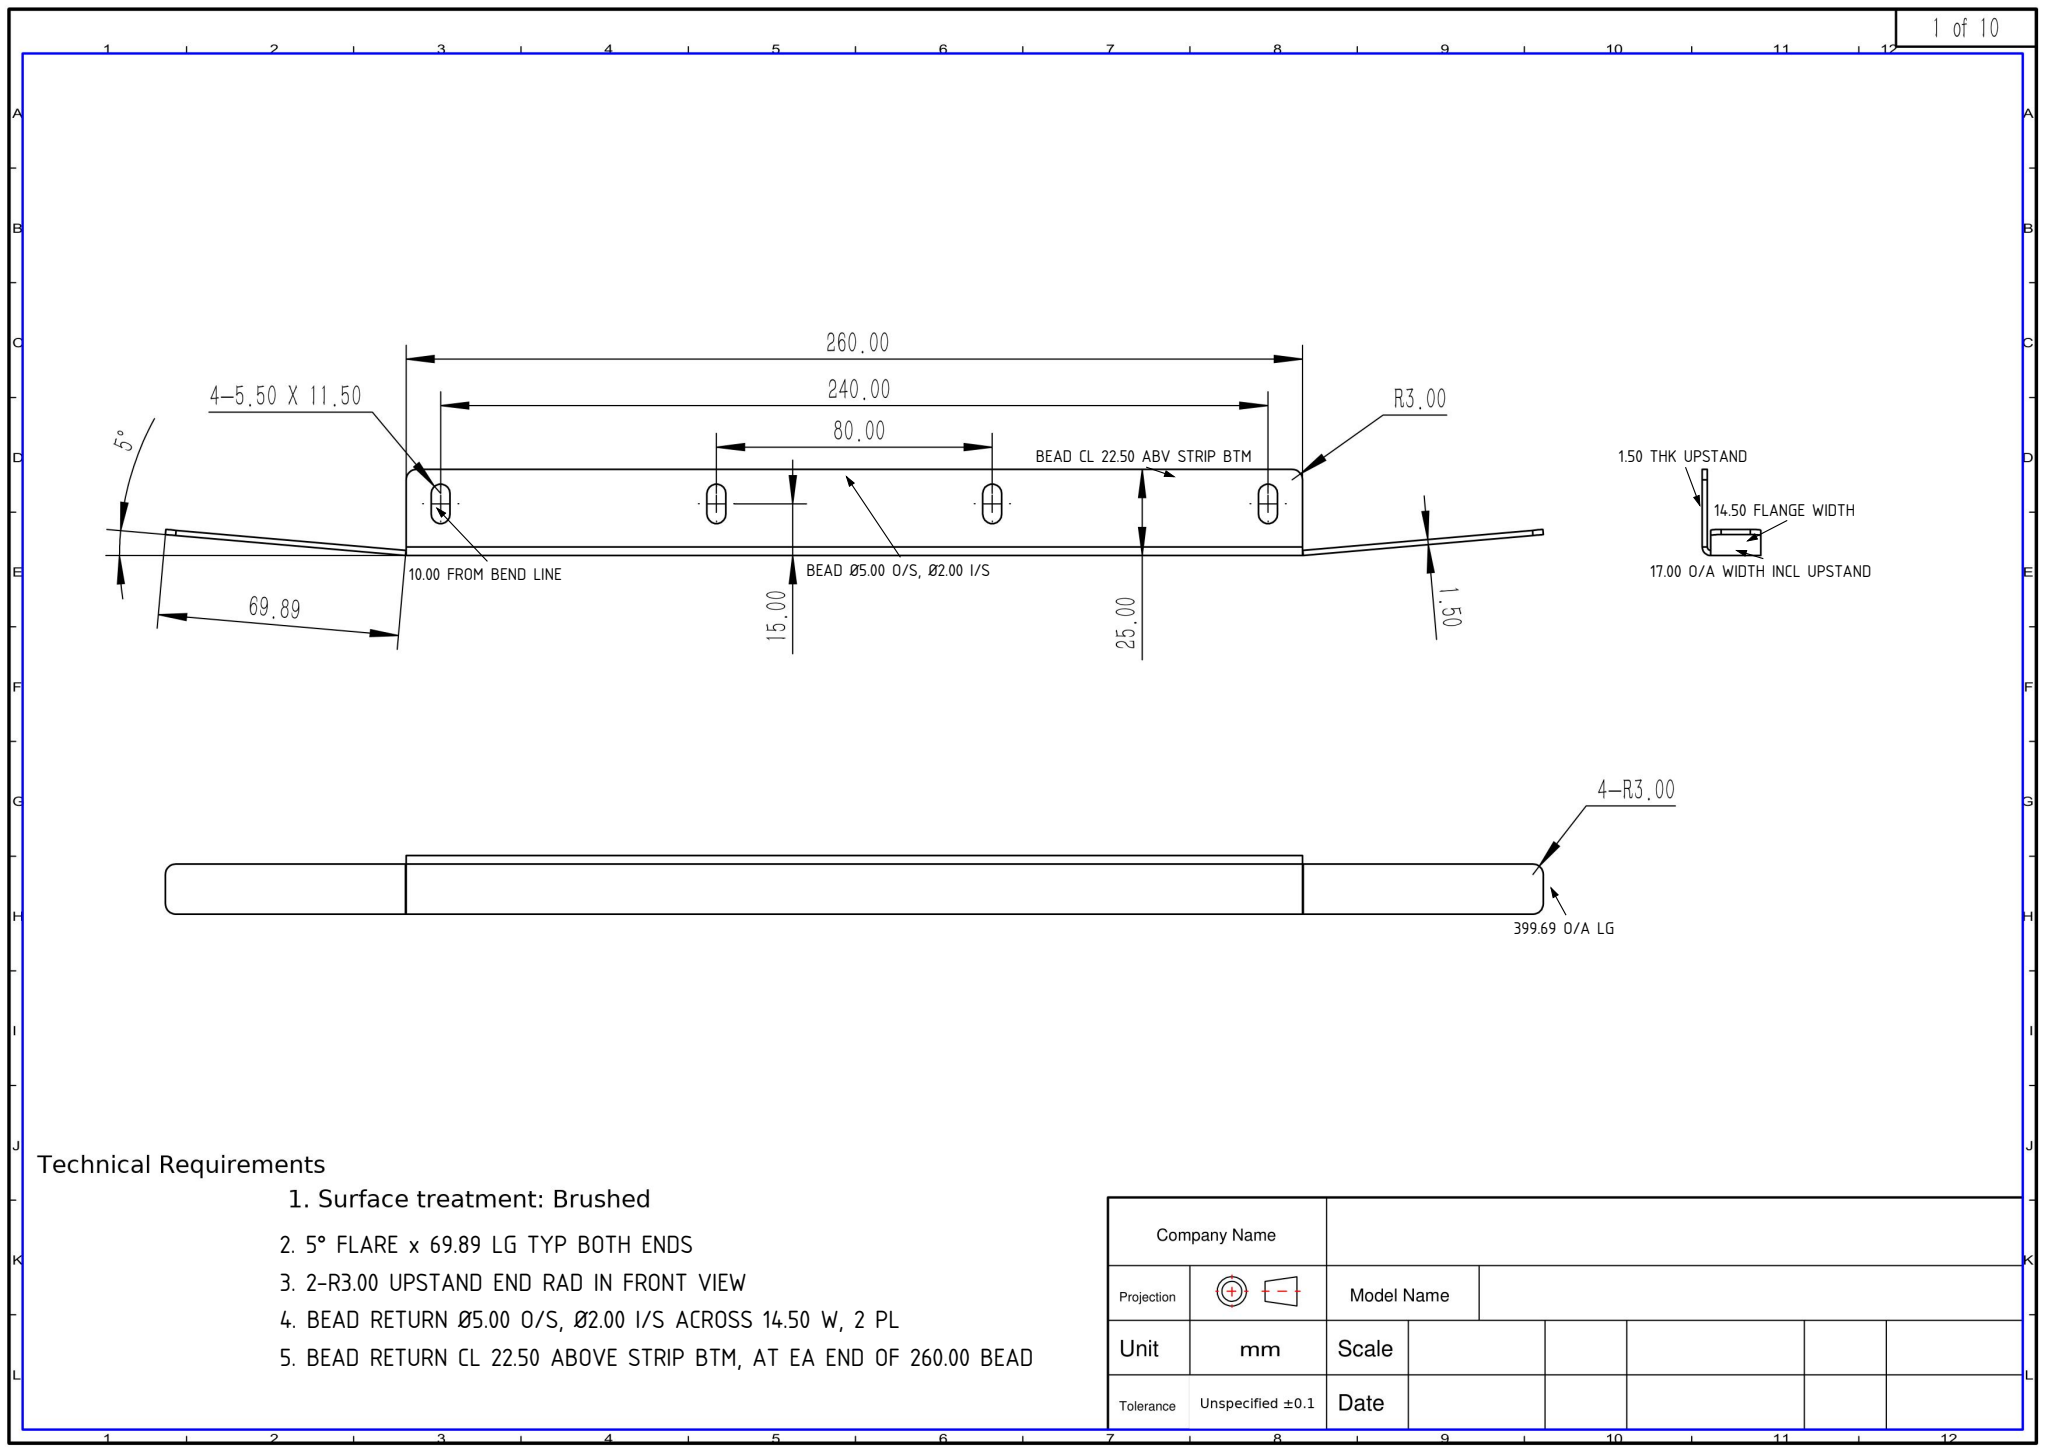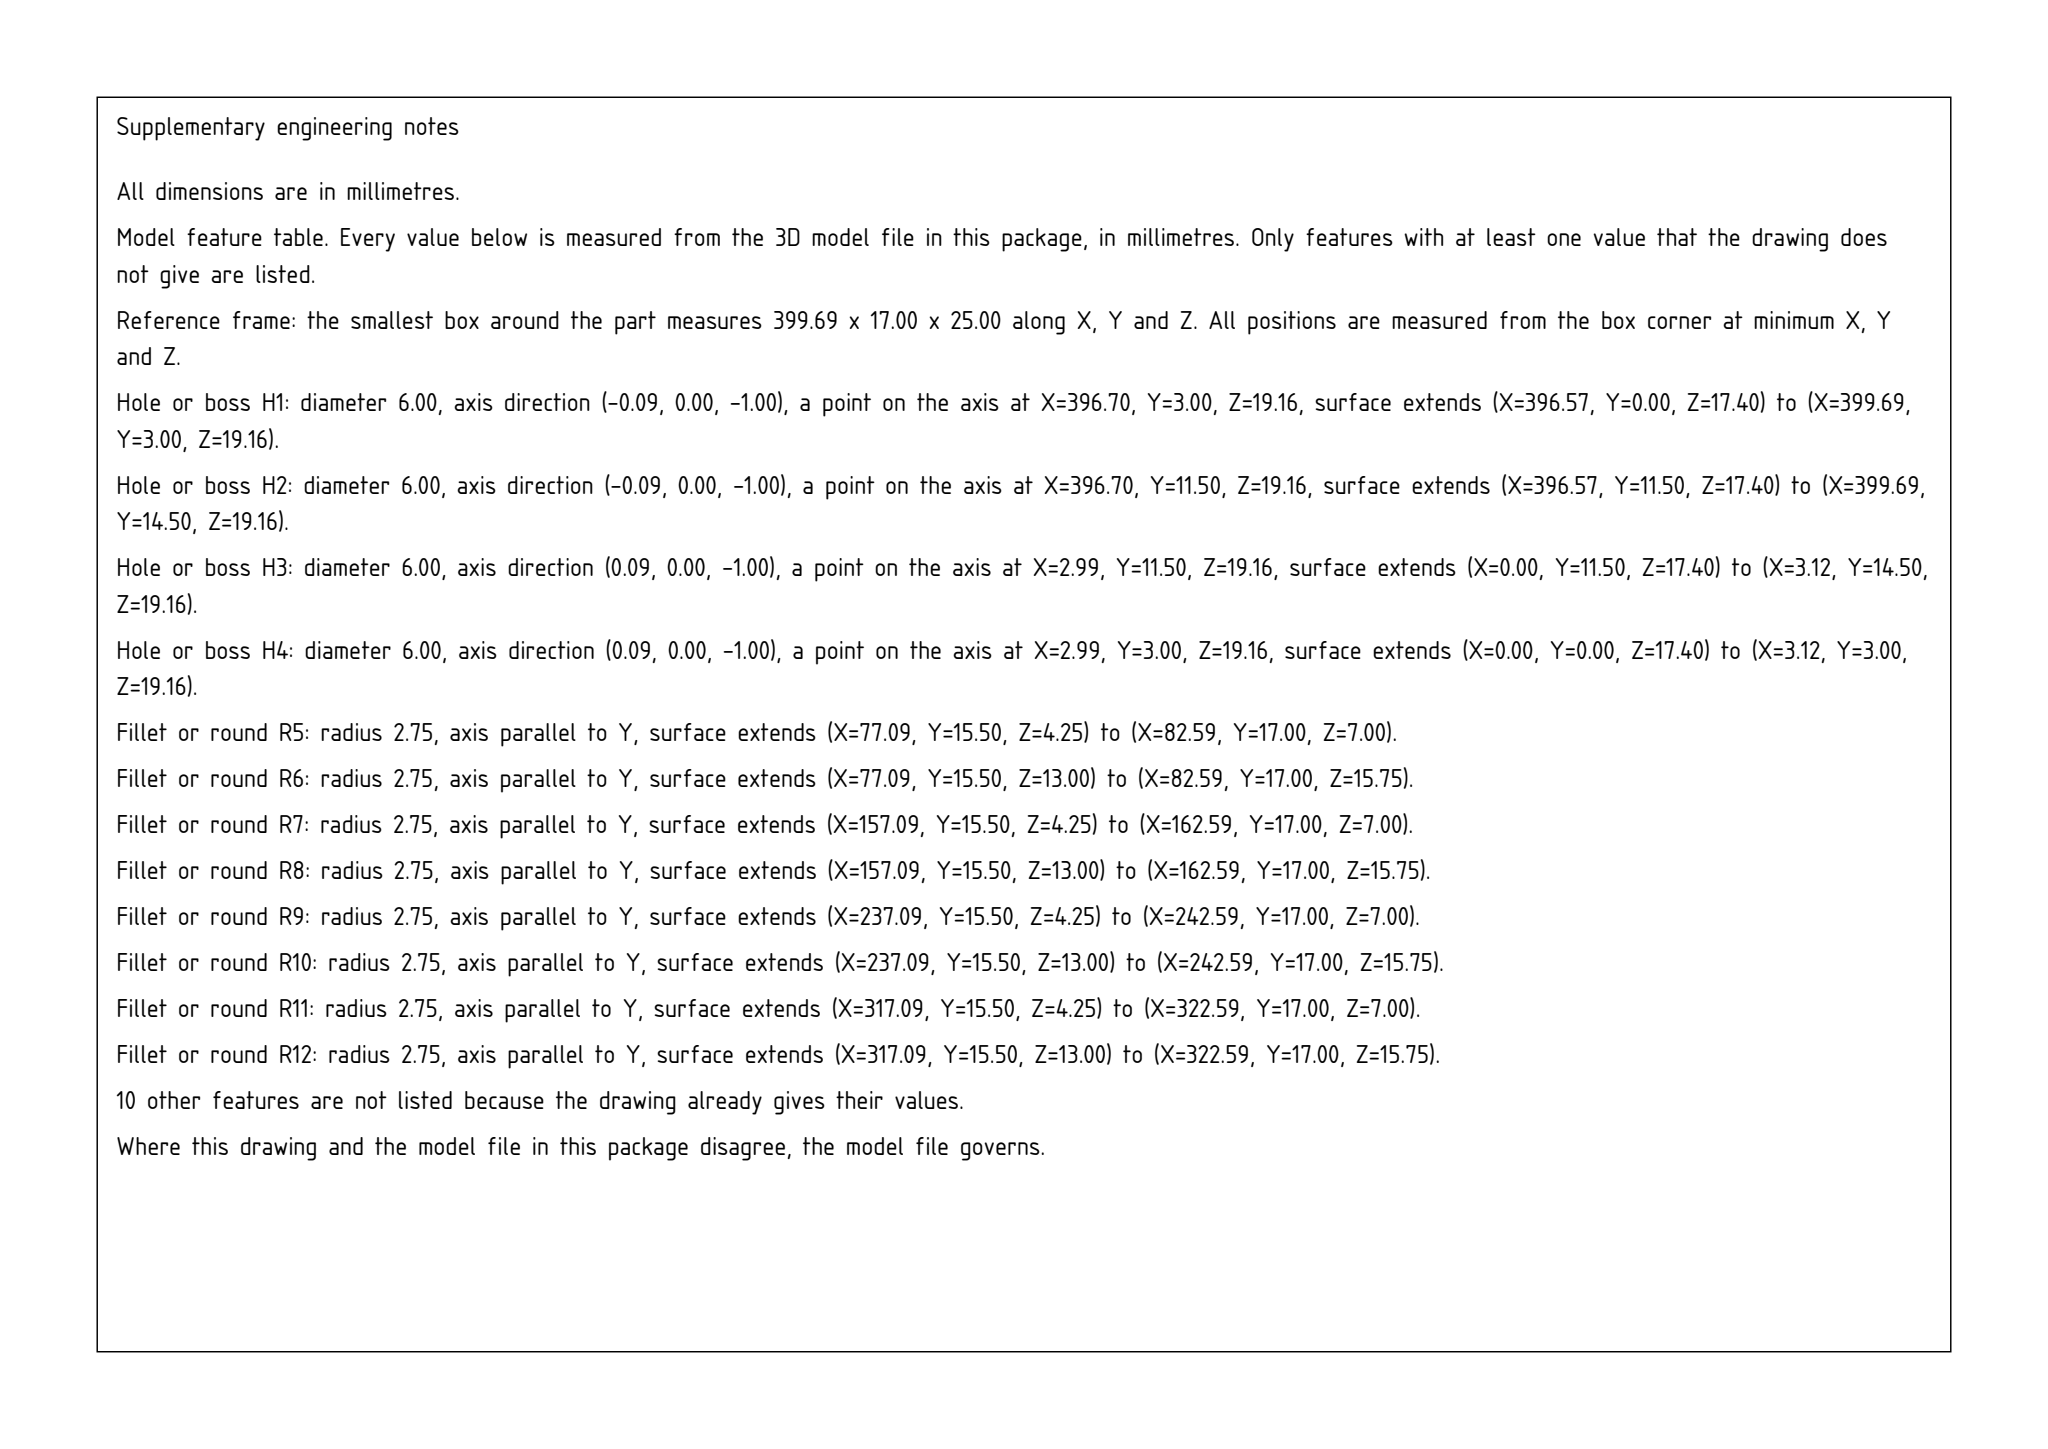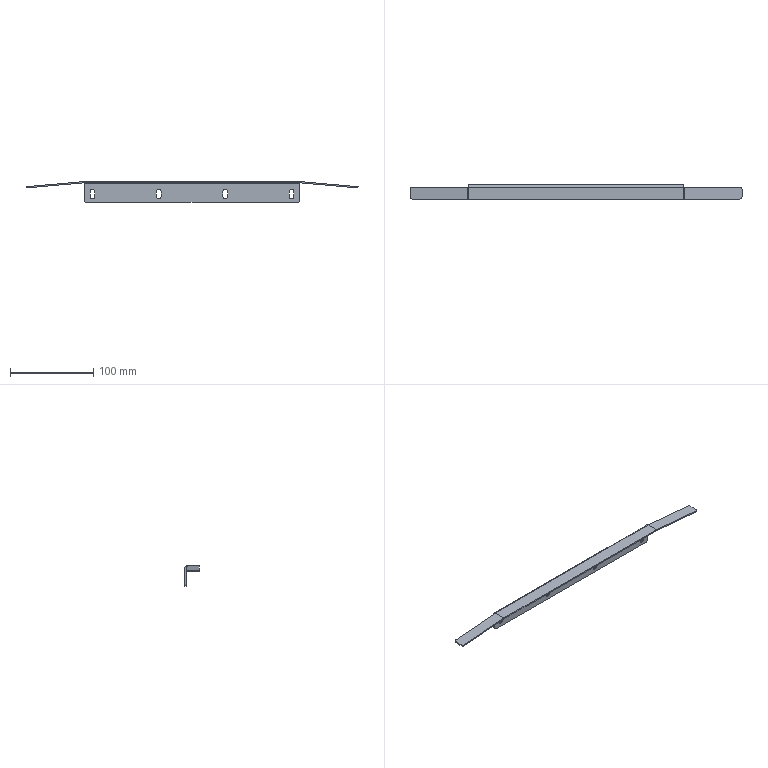Part | SolidWorks | mm | 1 solid | 56 faces | box 399.69 x 17 x 25 mm | volume 18191 mm3 | plane 32 | cylinder 24 | commonest cylinder face diameters 5.5 x12 6 x6 5 x3 2 x3
Drawing notes:
PLAN: 17.00 O/A WIDTH INCL UPSTAND | from the solid: bbox_xyz y=17.0
FLAT STRIP/FLANGE WIDTH 14.50 (EXCL UPSTAND) | from the solid: y planes at 0.0 and 14.5 bounding flange
UPSTAND 1.50 THK; WALL FACES 15.50 & 17.00 FROM STRIP EDGE | from the solid: y planes at 15.5 and 17.0, datum y=0 strip edge
1ST SLOT CL 10.00 FROM BEND LINE; 4 SLOTS @ 80.00 PITCH TYP | from the solid: Bend/upstand plane x=69.84; slot ctrs x=79.84,159.84,239.84,319.84 (Ø5.5)
ROLLED BEAD ON UPSTAND EDGE: O/S Ø5.00, I/S Ø2.00, L260.00 | from the solid: Coaxial cylinders dia 5.0 & 2.0, axis x, pos (y14.5, z22.5), L260.0
BEAD CL 2.50 FROM UPSTAND O/S FACE, 22.50 ABOVE STRIP BOT FACE | from the solid: Bead axis y=14.5, z=22.5; outer face y=17.0; z planes 0.0 and 25.0
OVERALL LENGTH 399.69 | from the solid: bbox_xyz x = 399.686
5° FLARE x 69.89 LG TYP BOTH ENDS | from the solid: upstand ends at x=69.84 & 329.84; 260.00 flat between, 69.84 each end
2-R3.00 UPSTAND END RAD IN FRONT VIEW | from the solid: R3 upstand ends at x=69.84 and x=329.84 (2 pl)
BEAD RETURN Ø5.00 O/S, Ø2.00 I/S ACROSS 14.50 W, 2 PL | from the solid: cyl dia 5.0 & 2.0, axis y, len 14.5 at x=69.84 and x=329.84
BEAD RETURN CL 22.50 ABOVE STRIP BTM, AT EA END OF 260.00 BEAD | from the solid: y-axis bead cyls pos z=22.5; x=69.84 & 329.84 = ends of 260.00 bead